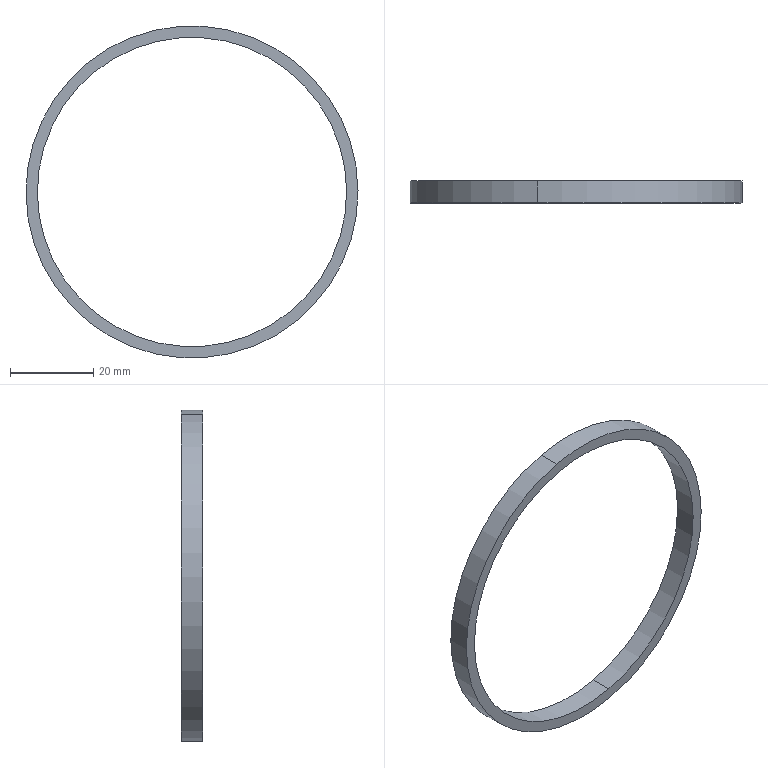Component | SolidWorks | 16-1 | 1 solid | 6 faces | box 80 x 5.3 x 80 mm | volume 3525 mm3 | cylinder 4 | plane 2 | commonest cylinder face diameters 74.52 x2 80 x2
build123d program:
from build123d import *

# Parameters (mm, degrees)
SKETCH1_R           = 40
SKETCH1_R_2         = 37.26
BOSS_EXTRUDE1_DEPTH = 5.3


with BuildPart() as part:
    # Sketch1 → Boss-Extrude1 (new body)
    with BuildSketch(Plane(origin=(0, 0, 0), x_dir=(1, 0, 0), z_dir=(0, 1, 0))):
        with Locations(Location((0, 0, 0), (0, 0, 270))):
            Circle(SKETCH1_R)
        with Locations(Location((0, 0, 0), (0, 0, 270))):
            Circle(SKETCH1_R_2, mode=Mode.SUBTRACT)
    extrude(amount=BOSS_EXTRUDE1_DEPTH)


solid = part.part

# Placed as in the assembly
solid = solid.moved(Location((0, -3.3, 0), (0, 0, 0)))
STEP:
#1=COLOUR_RGB('',0.7922,0.8196,0.9333);
#2=FILL_AREA_STYLE_COLOUR('',#1);
#3=FILL_AREA_STYLE('',(#2));
#4=SURFACE_STYLE_FILL_AREA(#3);
#5=SURFACE_SIDE_STYLE('',(#4));
#6=SURFACE_STYLE_USAGE(.BOTH.,#5);
#7=PRESENTATION_STYLE_ASSIGNMENT((#6));
#8=CARTESIAN_POINT('',(0.3375,0.07874,-1.428));
#9=VERTEX_POINT('',#8);
#10=CARTESIAN_POINT('',(-0.3375,0.07874,1.428));
#11=VERTEX_POINT('',#10);
#12=CARTESIAN_POINT('',(0.,0.07874,0.));
#13=DIRECTION('',(0.,1.,0.));
#14=DIRECTION('',(-0.2301,0.,0.9732));
#15=AXIS2_PLACEMENT_3D('',#12,#13,#14);
#16=CIRCLE('',#15,1.467);
#17=EDGE_CURVE('',#9,#11,#16,.T.);
#18=ORIENTED_EDGE('',*,*,#17,.T.);
#19=CARTESIAN_POINT('',(-0.3375,-0.1299,1.428));
#20=VERTEX_POINT('',#19);
#21=CARTESIAN_POINT('',(-0.3375,0.07874,1.428));
#22=DIRECTION('',(0.,-1.,0.));
#23=VECTOR('',#22,39.37);
#24=LINE('',#21,#23);
#25=EDGE_CURVE('',#11,#20,#24,.T.);
#26=ORIENTED_EDGE('',*,*,#25,.T.);
#27=CARTESIAN_POINT('',(0.3375,-0.1299,-1.428));
#28=VERTEX_POINT('',#27);
#29=CARTESIAN_POINT('',(0.,-0.1299,0.));
#30=DIRECTION('',(0.,1.,0.));
#31=DIRECTION('',(-0.2301,0.,0.9732));
#32=AXIS2_PLACEMENT_3D('',#29,#30,#31);
#33=CIRCLE('',#32,1.467);
#34=EDGE_CURVE('',#28,#20,#33,.T.);
#35=ORIENTED_EDGE('',*,*,#34,.F.);
#36=CARTESIAN_POINT('',(0.3375,0.07874,-1.428));
#37=DIRECTION('',(0.,-1.,0.));
#38=VECTOR('',#37,39.37);
#39=LINE('',#36,#38);
#40=EDGE_CURVE('',#9,#28,#39,.T.);
#41=ORIENTED_EDGE('',*,*,#40,.F.);
#42=EDGE_LOOP('',(#18,#26,#35,#41));
#43=FACE_OUTER_BOUND('',#42,.T.);
#44=CARTESIAN_POINT('',(0.,0.07874,0.));
#45=DIRECTION('',(0.,-1.,0.));
#46=DIRECTION('',(0.2301,0.,-0.9732));
#47=AXIS2_PLACEMENT_3D('',#44,#45,#46);
#48=CYLINDRICAL_SURFACE('',#47,1.467);
#49=ADVANCED_FACE('',(#43),#48,.F.);
#50=CARTESIAN_POINT('',(-0.3623,0.07874,1.533));
#51=VERTEX_POINT('',#50);
#52=CARTESIAN_POINT('',(0.3623,0.07874,-1.533));
#53=VERTEX_POINT('',#52);
#54=CARTESIAN_POINT('',(0.,0.07874,0.));
#55=DIRECTION('',(0.,1.,0.));
#56=DIRECTION('',(-0.2301,0.,0.9732));
#57=AXIS2_PLACEMENT_3D('',#54,#55,#56);
#58=CIRCLE('',#57,1.575);
#59=EDGE_CURVE('',#51,#53,#58,.T.);
#60=ORIENTED_EDGE('',*,*,#59,.F.);
#61=CARTESIAN_POINT('',(-0.3623,-0.1299,1.533));
#62=VERTEX_POINT('',#61);
#63=CARTESIAN_POINT('',(-0.3623,0.07874,1.533));
#64=DIRECTION('',(0.,-1.,0.));
#65=VECTOR('',#64,39.37);
#66=LINE('',#63,#65);
#67=EDGE_CURVE('',#51,#62,#66,.T.);
#68=ORIENTED_EDGE('',*,*,#67,.T.);
#69=CARTESIAN_POINT('',(0.3623,-0.1299,-1.533));
#70=VERTEX_POINT('',#69);
#71=CARTESIAN_POINT('',(0.,-0.1299,0.));
#72=DIRECTION('',(0.,1.,0.));
#73=DIRECTION('',(-0.2301,0.,0.9732));
#74=AXIS2_PLACEMENT_3D('',#71,#72,#73);
#75=CIRCLE('',#74,1.575);
#76=EDGE_CURVE('',#62,#70,#75,.T.);
#77=ORIENTED_EDGE('',*,*,#76,.T.);
#78=CARTESIAN_POINT('',(0.3623,0.07874,-1.533));
#79=DIRECTION('',(0.,-1.,0.));
#80=VECTOR('',#79,39.37);
#81=LINE('',#78,#80);
#82=EDGE_CURVE('',#53,#70,#81,.T.);
#83=ORIENTED_EDGE('',*,*,#82,.F.);
#84=EDGE_LOOP('',(#60,#68,#77,#83));
#85=FACE_OUTER_BOUND('',#84,.T.);
#86=CARTESIAN_POINT('',(0.,0.07874,0.));
#87=DIRECTION('',(0.,-1.,0.));
#88=DIRECTION('',(0.2301,0.,-0.9732));
#89=AXIS2_PLACEMENT_3D('',#86,#87,#88);
#90=CYLINDRICAL_SURFACE('',#89,1.575);
#91=ADVANCED_FACE('',(#85),#90,.T.);
#92=CARTESIAN_POINT('',(0.,0.07874,0.));
#93=DIRECTION('',(0.,1.,0.));
#94=DIRECTION('',(-0.2301,0.,0.9732));
#95=AXIS2_PLACEMENT_3D('',#92,#93,#94);
#96=CIRCLE('',#95,1.575);
#97=EDGE_CURVE('',#53,#51,#96,.T.);
#98=ORIENTED_EDGE('',*,*,#97,.T.);
#99=ORIENTED_EDGE('',*,*,#59,.T.);
#100=EDGE_LOOP('',(#98,#99));
#101=FACE_OUTER_BOUND('',#100,.T.);
#102=ORIENTED_EDGE('',*,*,#17,.F.);
#103=CARTESIAN_POINT('',(0.,0.07874,0.));
#104=DIRECTION('',(0.,1.,0.));
#105=DIRECTION('',(-0.2301,0.,0.9732));
#106=AXIS2_PLACEMENT_3D('',#103,#104,#105);
#107=CIRCLE('',#106,1.467);
#108=EDGE_CURVE('',#11,#9,#107,.T.);
#109=ORIENTED_EDGE('',*,*,#108,.F.);
#110=EDGE_LOOP('',(#102,#109));
#111=FACE_BOUND('',#110,.T.);
#112=CARTESIAN_POINT('',(0.,0.07874,0.));
#113=DIRECTION('',(0.,1.,0.));
#114=DIRECTION('',(-0.2301,0.,0.9732));
#115=AXIS2_PLACEMENT_3D('',#112,#113,#114);
#116=PLANE('',#115);
#117=ADVANCED_FACE('',(#101,#111),#116,.T.);
#118=CARTESIAN_POINT('',(0.,-0.1299,0.));
#119=DIRECTION('',(0.,1.,0.));
#120=DIRECTION('',(-0.2301,0.,0.9732));
#121=AXIS2_PLACEMENT_3D('',#118,#119,#120);
#122=CIRCLE('',#121,1.575);
#123=EDGE_CURVE('',#70,#62,#122,.T.);
#124=ORIENTED_EDGE('',*,*,#123,.F.);
#125=ORIENTED_EDGE('',*,*,#76,.F.);
#126=EDGE_LOOP('',(#124,#125));
#127=FACE_OUTER_BOUND('',#126,.T.);
#128=ORIENTED_EDGE('',*,*,#34,.T.);
#129=CARTESIAN_POINT('',(0.,-0.1299,0.));
#130=DIRECTION('',(0.,1.,0.));
#131=DIRECTION('',(-0.2301,0.,0.9732));
#132=AXIS2_PLACEMENT_3D('',#129,#130,#131);
#133=CIRCLE('',#132,1.467);
#134=EDGE_CURVE('',#20,#28,#133,.T.);
#135=ORIENTED_EDGE('',*,*,#134,.T.);
#136=EDGE_LOOP('',(#128,#135));
#137=FACE_BOUND('',#136,.T.);
#138=CARTESIAN_POINT('',(0.,-0.1299,0.));
#139=DIRECTION('',(0.,1.,0.));
#140=DIRECTION('',(-0.2301,0.,0.9732));
#141=AXIS2_PLACEMENT_3D('',#138,#139,#140);
#142=PLANE('',#141);
#143=ADVANCED_FACE('',(#127,#137),#142,.F.);
#144=ORIENTED_EDGE('',*,*,#67,.F.);
#145=ORIENTED_EDGE('',*,*,#97,.F.);
#146=ORIENTED_EDGE('',*,*,#82,.T.);
#147=ORIENTED_EDGE('',*,*,#123,.T.);
#148=EDGE_LOOP('',(#144,#145,#146,#147));
#149=FACE_OUTER_BOUND('',#148,.T.);
#150=CARTESIAN_POINT('',(0.,0.07874,0.));
#151=DIRECTION('',(0.,-1.,0.));
#152=DIRECTION('',(0.2301,0.,-0.9732));
#153=AXIS2_PLACEMENT_3D('',#150,#151,#152);
#154=CYLINDRICAL_SURFACE('',#153,1.575);
#155=ADVANCED_FACE('',(#149),#154,.T.);
#156=ORIENTED_EDGE('',*,*,#25,.F.);
#157=ORIENTED_EDGE('',*,*,#108,.T.);
#158=ORIENTED_EDGE('',*,*,#40,.T.);
#159=ORIENTED_EDGE('',*,*,#134,.F.);
#160=EDGE_LOOP('',(#156,#157,#158,#159));
#161=FACE_OUTER_BOUND('',#160,.T.);
#162=CARTESIAN_POINT('',(0.,0.07874,0.));
#163=DIRECTION('',(0.,-1.,0.));
#164=DIRECTION('',(0.2301,0.,-0.9732));
#165=AXIS2_PLACEMENT_3D('',#162,#163,#164);
#166=CYLINDRICAL_SURFACE('',#165,1.467);
#167=ADVANCED_FACE('',(#161),#166,.F.);
#168=CLOSED_SHELL('',(#49,#91,#117,#143,#155,#167));
#169=MANIFOLD_SOLID_BREP('',#168);
#170=STYLED_ITEM('',(#7),#169);
#171=(LENGTH_UNIT()NAMED_UNIT(*)SI_UNIT($,.METRE.));
#172=LENGTH_MEASURE_WITH_UNIT(LENGTH_MEASURE(0.0254),#171);
#173=DIMENSIONAL_EXPONENTS(1.,0.,0.,0.,0.,0.,0.);
#174=(CONVERSION_BASED_UNIT('',#172)LENGTH_UNIT()NAMED_UNIT(#173));
#175=UNCERTAINTY_MEASURE_WITH_UNIT(LENGTH_MEASURE(0.00001),#174,'','');
#176=(NAMED_UNIT(*)PLANE_ANGLE_UNIT()SI_UNIT($,.RADIAN.));
#177=(NAMED_UNIT(*)SI_UNIT($,.STERADIAN.)SOLID_ANGLE_UNIT());
#178=(GEOMETRIC_REPRESENTATION_CONTEXT(3)GLOBAL_UNCERTAINTY_ASSIGNED_CONTEXT((#175))GLOBAL_UNIT_ASSIGNED_CONTEXT((#174,#176,#177))REPRESENTATION_CONTEXT('',''));
#179=MECHANICAL_DESIGN_GEOMETRIC_PRESENTATION_REPRESENTATION('',(#170),#178);
#180=CARTESIAN_POINT('',(0.,0.,0.));
#181=DIRECTION('',(0.,0.,1.));
#182=DIRECTION('',(1.,0.,0.));
#183=AXIS2_PLACEMENT_3D('',#180,#181,#182);
#184=(LENGTH_UNIT()NAMED_UNIT(*)SI_UNIT($,.METRE.));
#185=LENGTH_MEASURE_WITH_UNIT(LENGTH_MEASURE(0.0254),#184);
#186=DIMENSIONAL_EXPONENTS(1.,0.,0.,0.,0.,0.,0.);
#187=(CONVERSION_BASED_UNIT('',#185)LENGTH_UNIT()NAMED_UNIT(#186));
#188=UNCERTAINTY_MEASURE_WITH_UNIT(LENGTH_MEASURE(0.00001),#187,'','');
#189=(NAMED_UNIT(*)PLANE_ANGLE_UNIT()SI_UNIT($,.RADIAN.));
#190=(NAMED_UNIT(*)SI_UNIT($,.STERADIAN.)SOLID_ANGLE_UNIT());
#191=(GEOMETRIC_REPRESENTATION_CONTEXT(3)GLOBAL_UNCERTAINTY_ASSIGNED_CONTEXT((#188))GLOBAL_UNIT_ASSIGNED_CONTEXT((#187,#189,#190))REPRESENTATION_CONTEXT('',''));
#192=ADVANCED_BREP_SHAPE_REPRESENTATION('',(#169,#183),#191);
#193=PRESENTATION_LAYER_ASSIGNMENT('','',(#170));